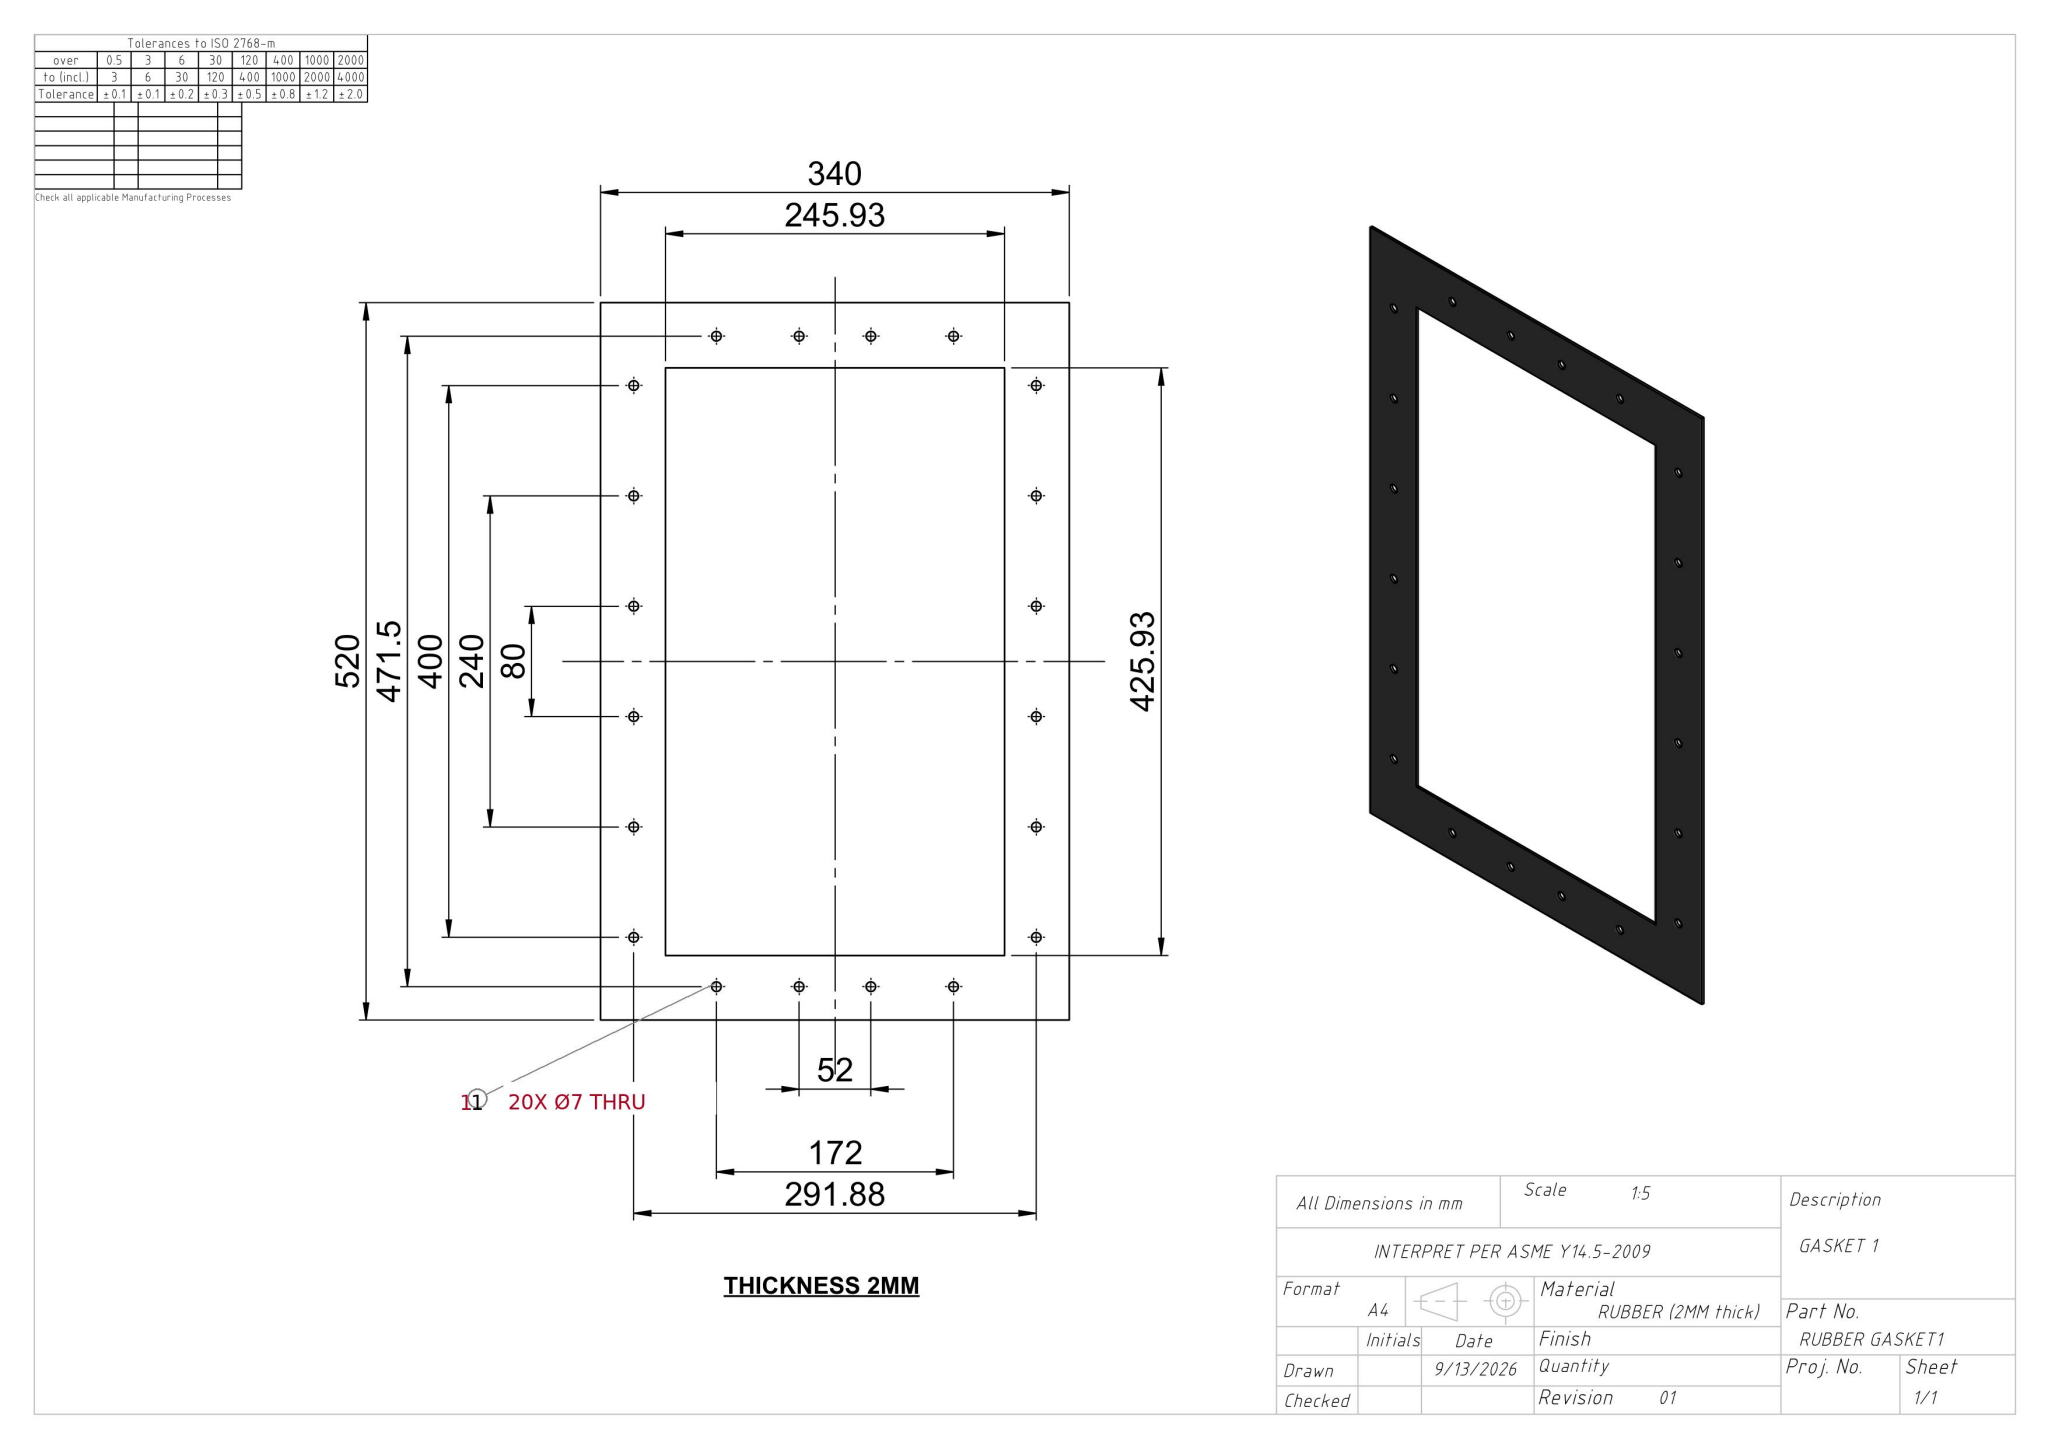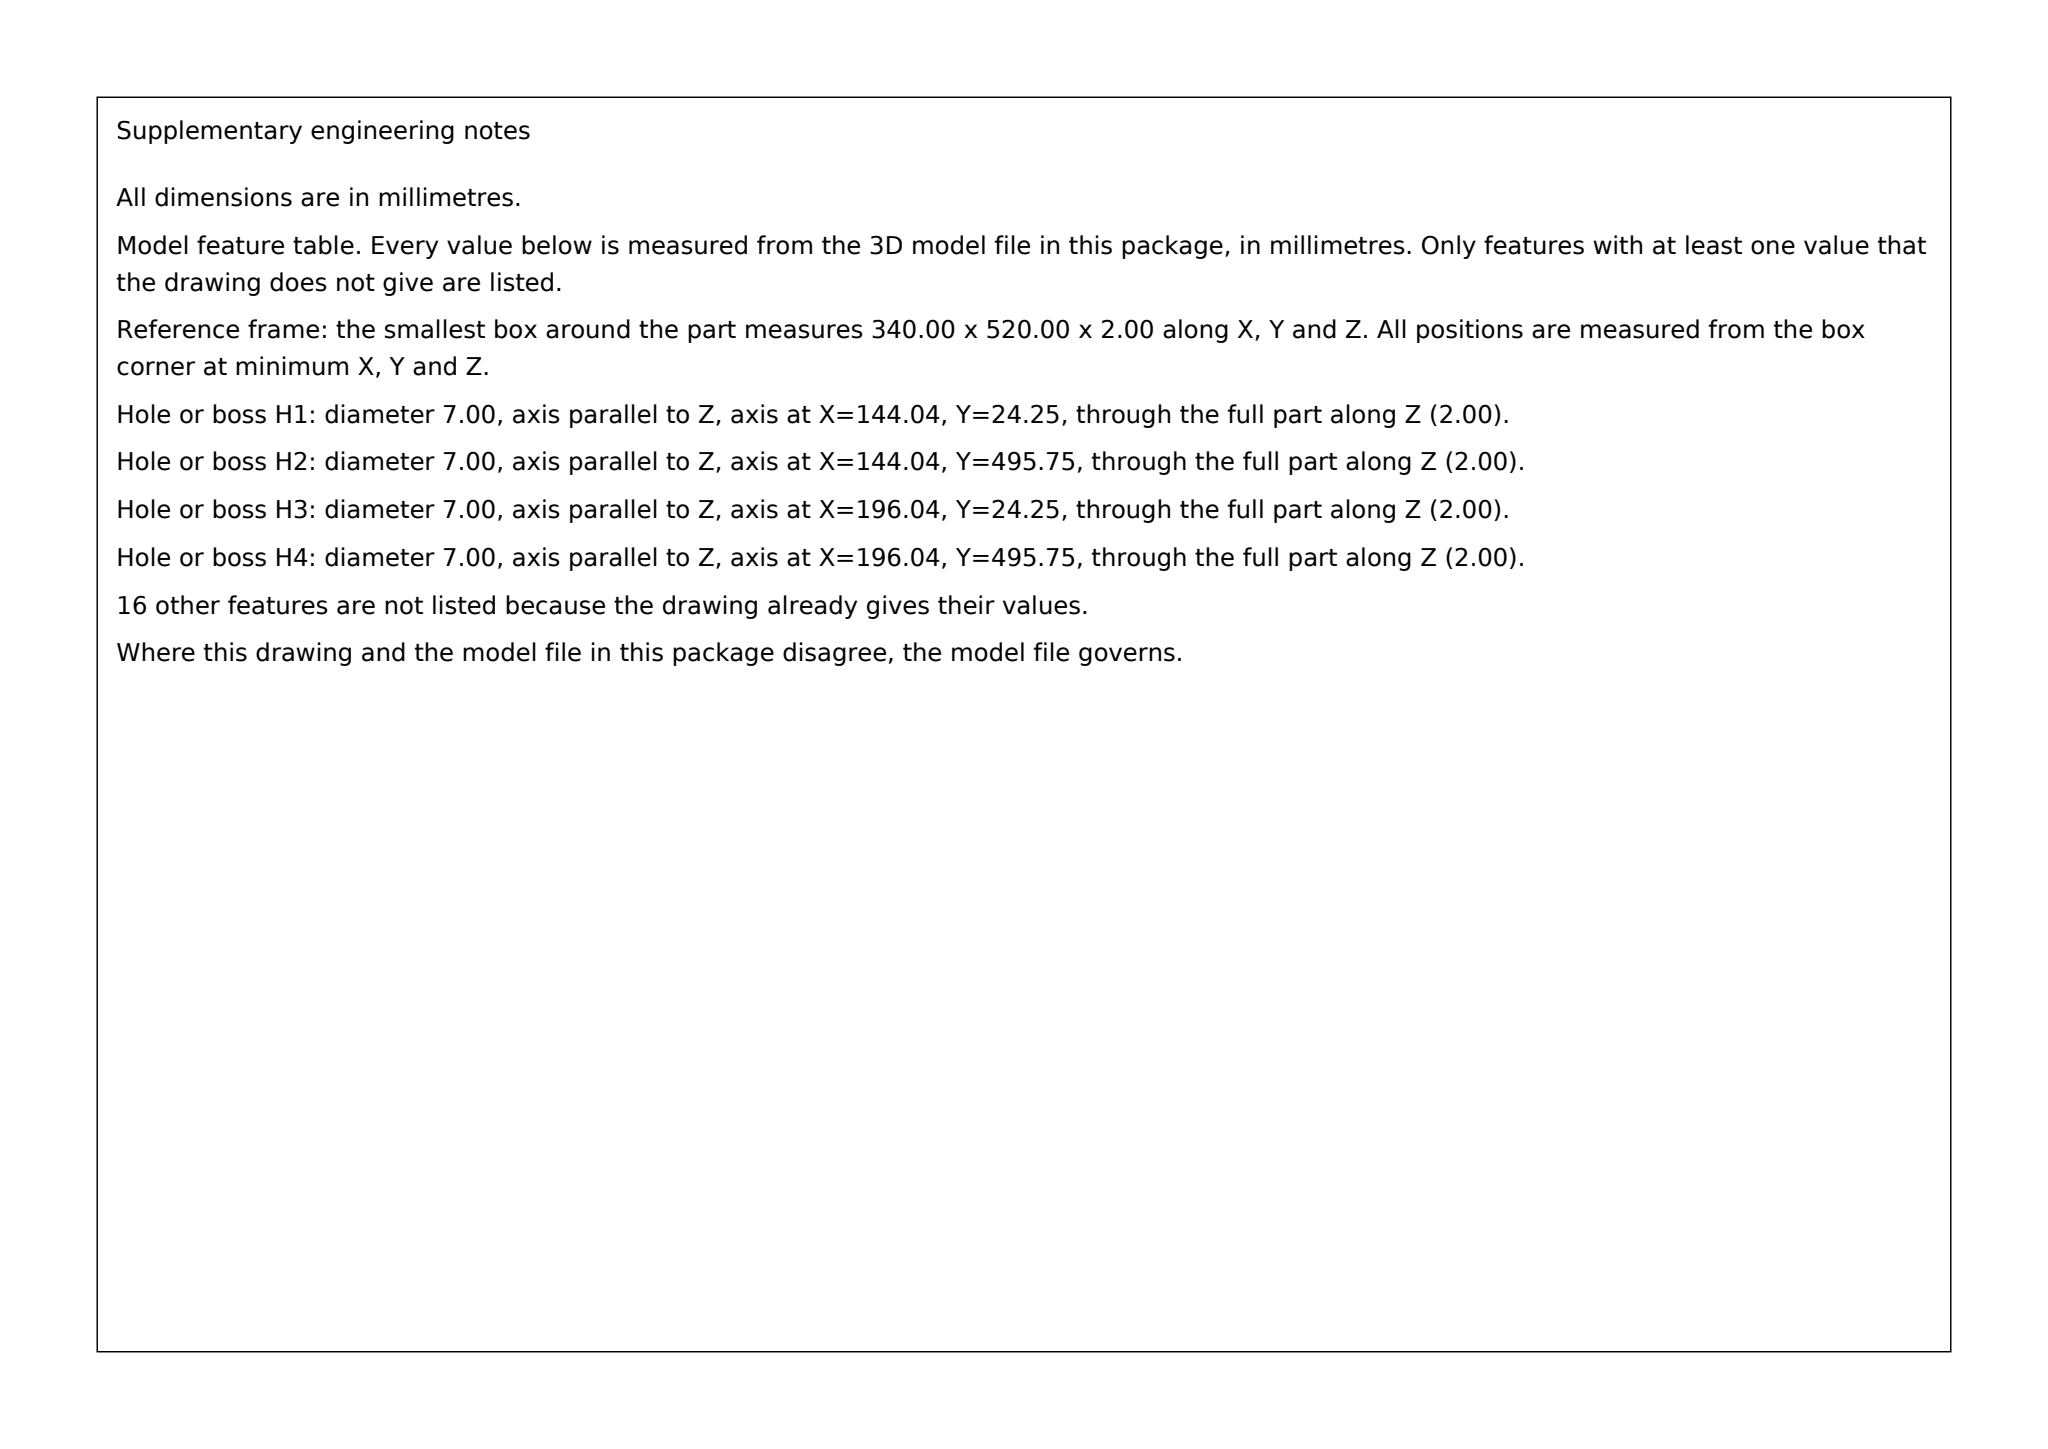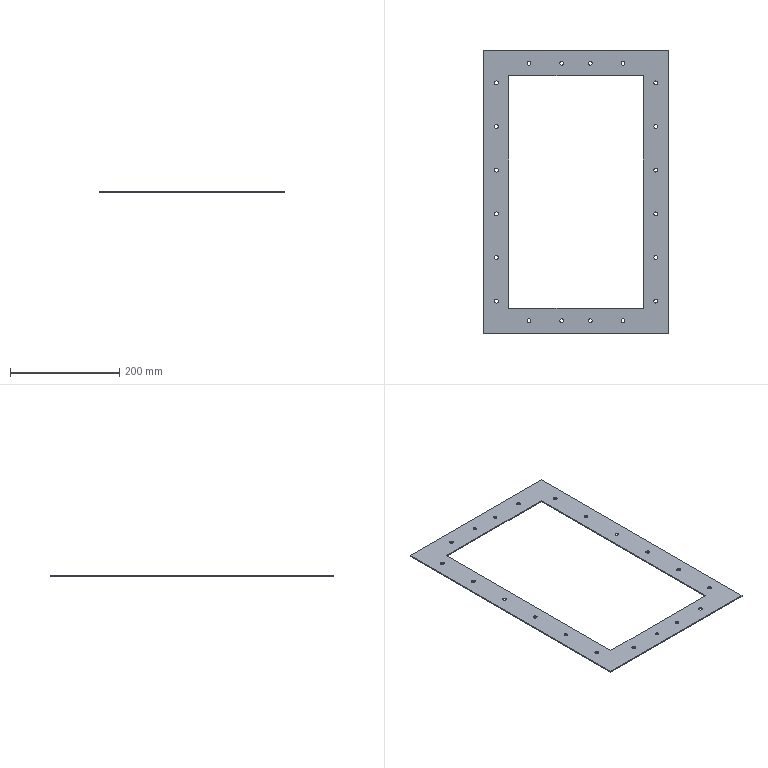Part | SolidWorks | mm | 1 solid | 50 faces | box 340 x 520 x 2 mm | volume 142564 mm3 | cylinder 40 | plane 10 | commonest cylinder face diameters 7 x40
build123d program:
from build123d import *

# Parameters (mm, degrees)
SKETCH1_W            = 340
SKETCH1_H            = 520
SKETCH1_W_2          = 245.929
SKETCH1_H_2          = 425.929
BOSS_EXTRUDE1_DEPTH  = 2
M6_CLEARANCE_HOLE1_D = 7


with BuildPart() as part:
    # Sketch1 → Boss-Extrude1 (new body)
    with BuildSketch(Plane.XY):
        with Locations((-0.03536, 1100.175)):
            Rectangle(SKETCH1_W, SKETCH1_H)
        with Locations((0.03536, 1100.035)):
            Rectangle(SKETCH1_W_2, SKETCH1_H_2, mode=Mode.SUBTRACT)
    extrude(amount=BOSS_EXTRUDE1_DEPTH)

    # M6 Clearance Hole1 (through all)
    with Locations(Plane(origin=(0, 0, 0), x_dir=(-1, 0, 0), z_dir=(0, 0, -1))):
        with Locations((-145.94, 900.175), (-86, 864.425), (-26, 864.425), (-145.94, 980.175), (-145.94, 1060.175), (-145.94, 1140.175), (-145.94, 1220.175), (-145.94, 1300.175), (-86, 1335.925), (-26, 1335.925), (26, 1335.925), (86, 1335.925), (145.94, 1300.175), (145.94, 1220.175), (145.94, 1140.175), (145.94, 1060.175), (145.94, 980.175), (26, 864.425), (86, 864.425), (145.94, 900.175)):
            Hole(M6_CLEARANCE_HOLE1_D / 2)


solid = part.part